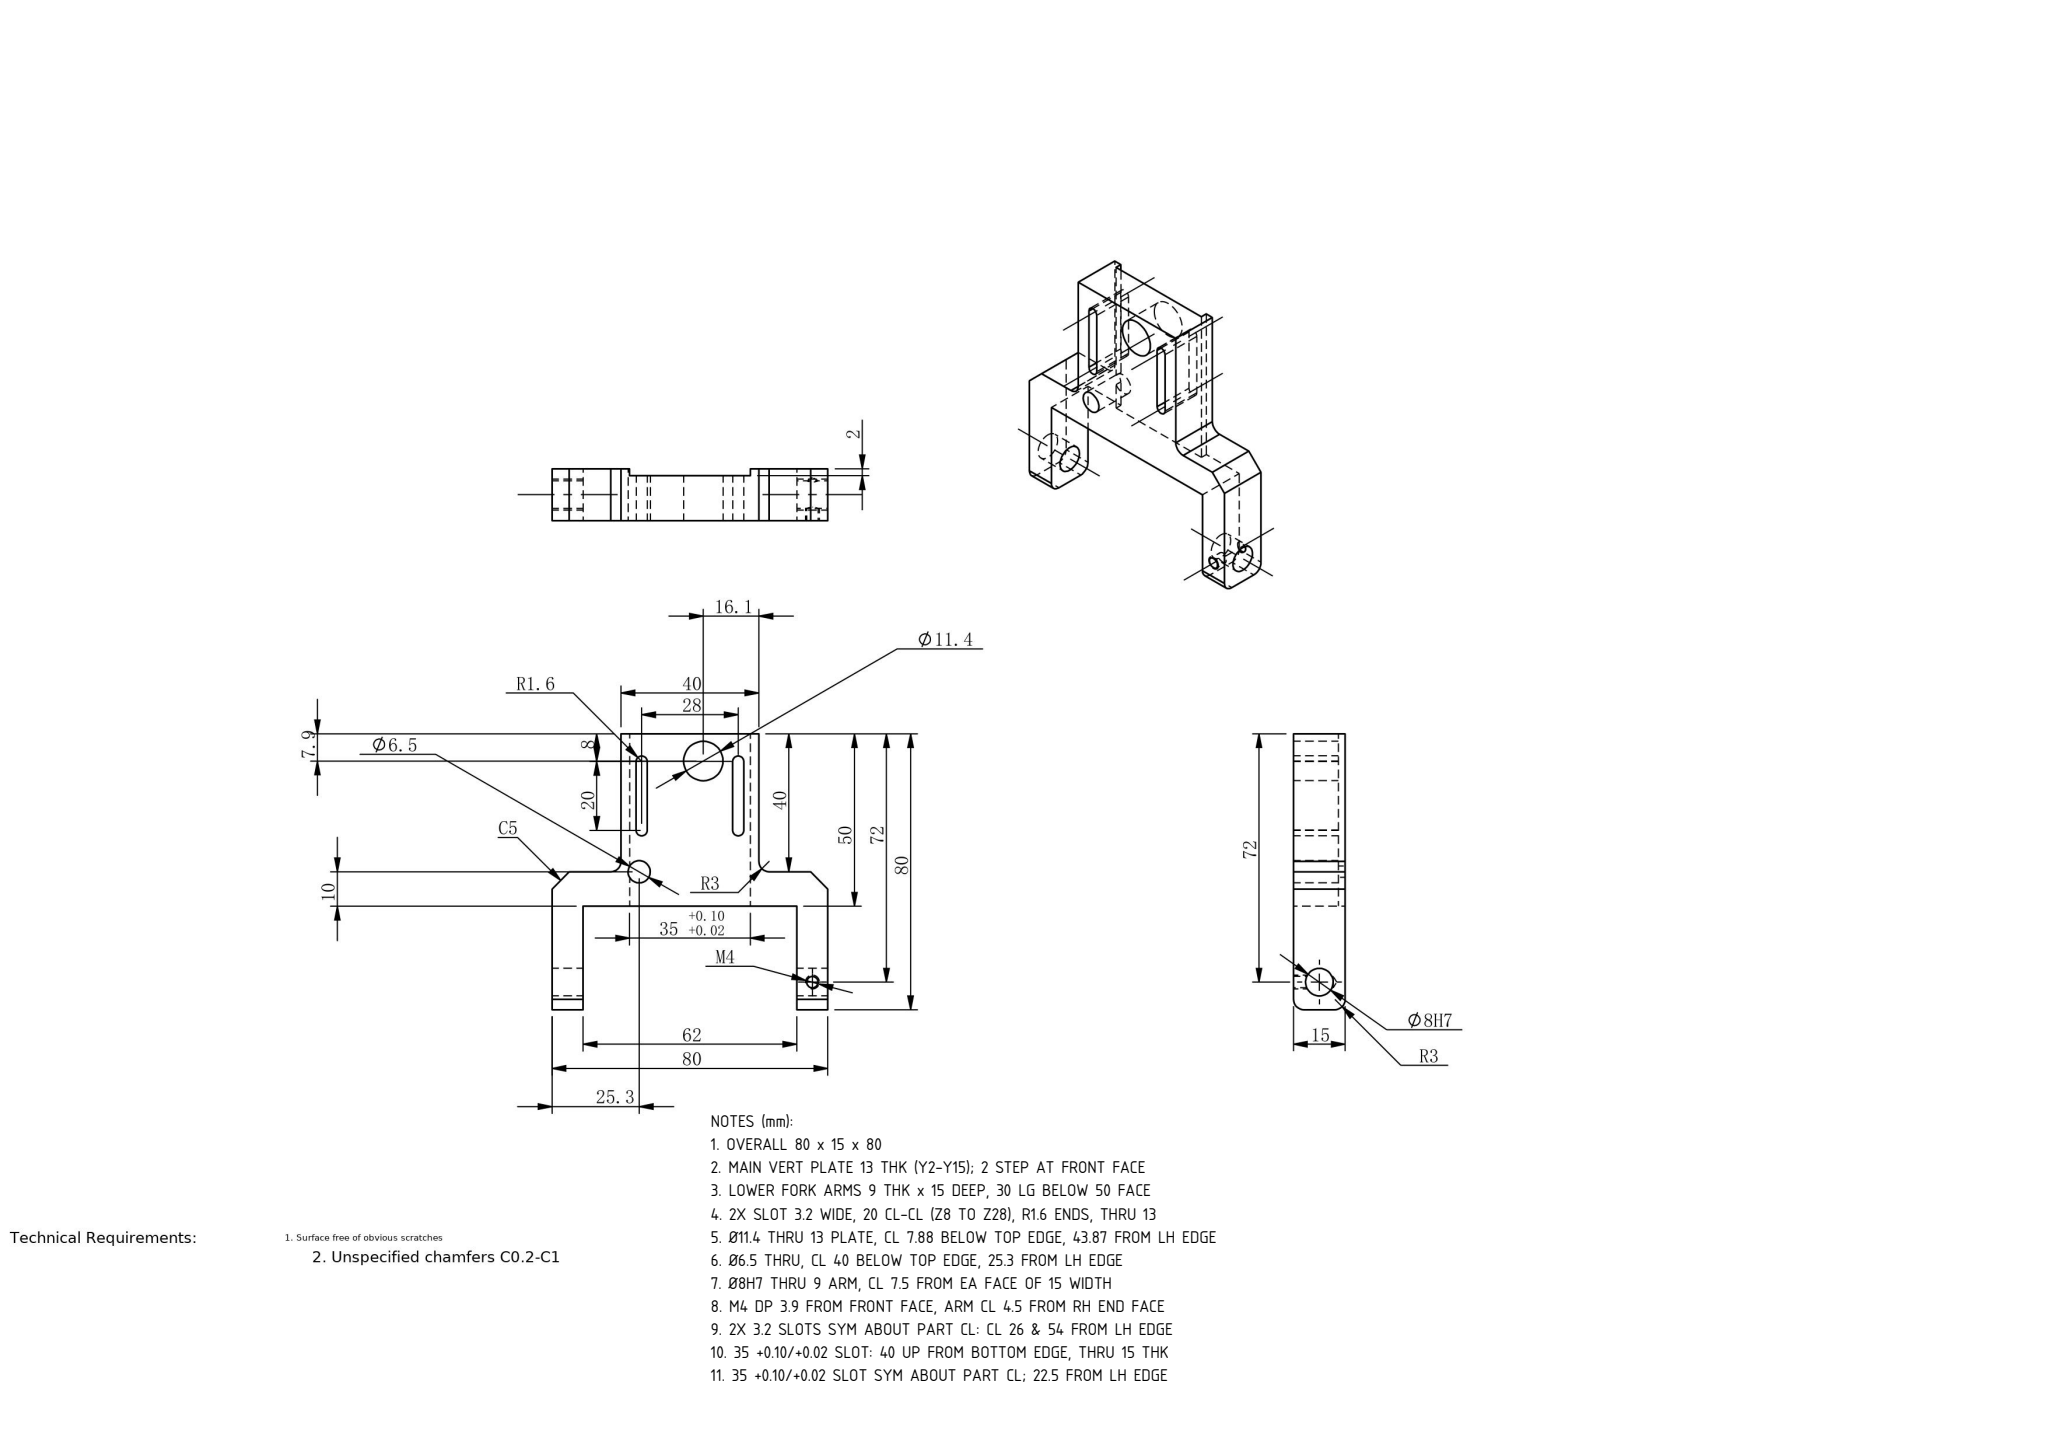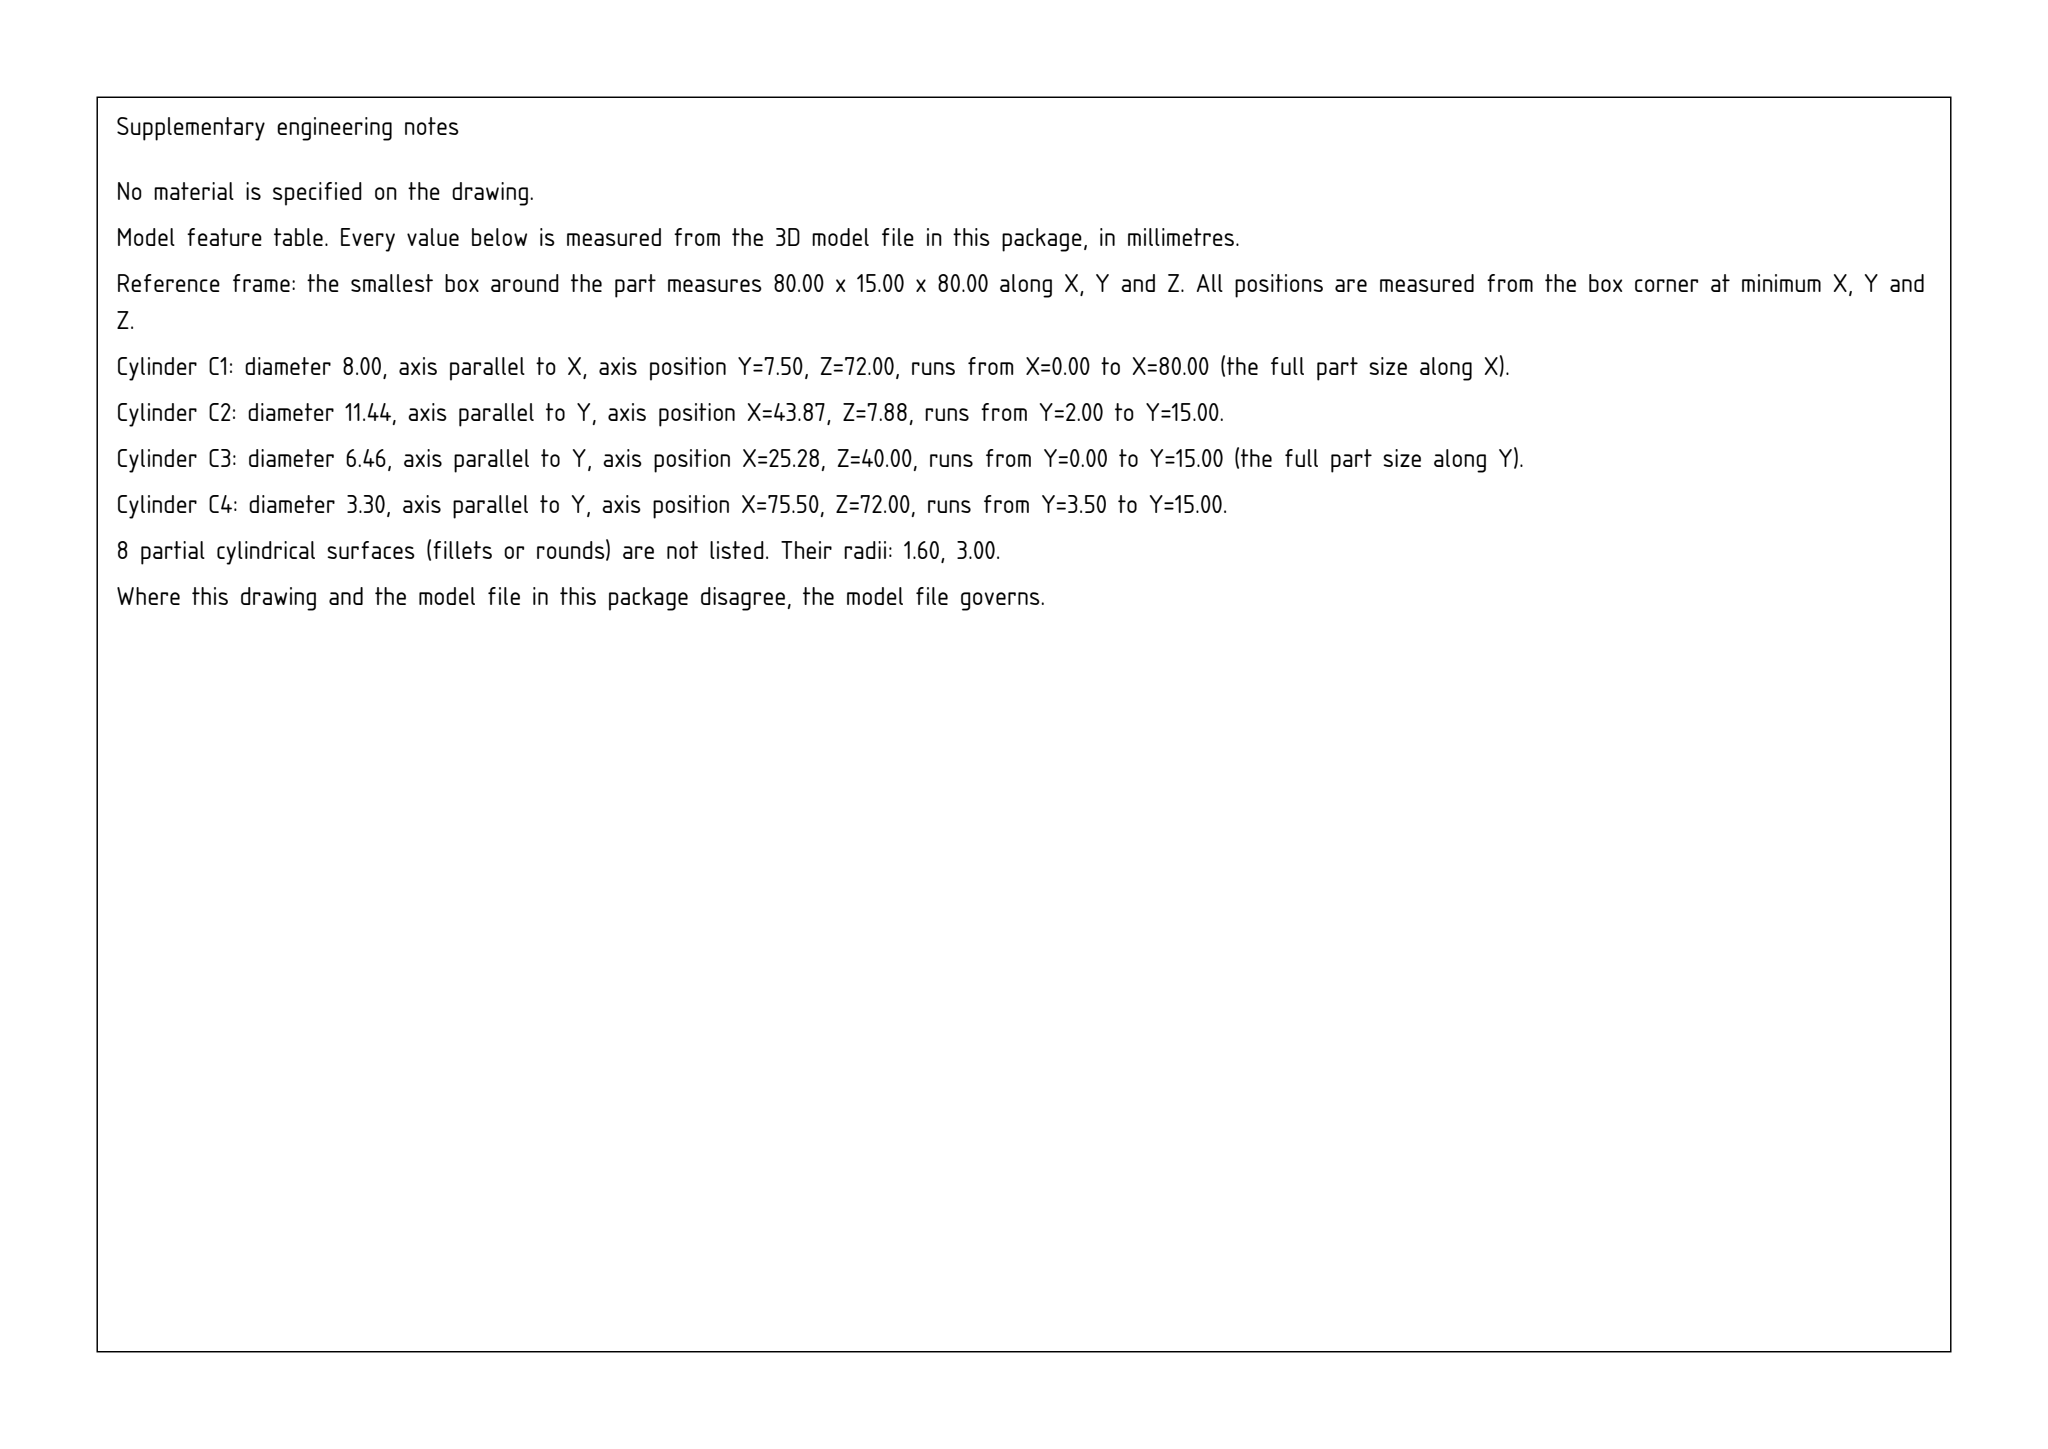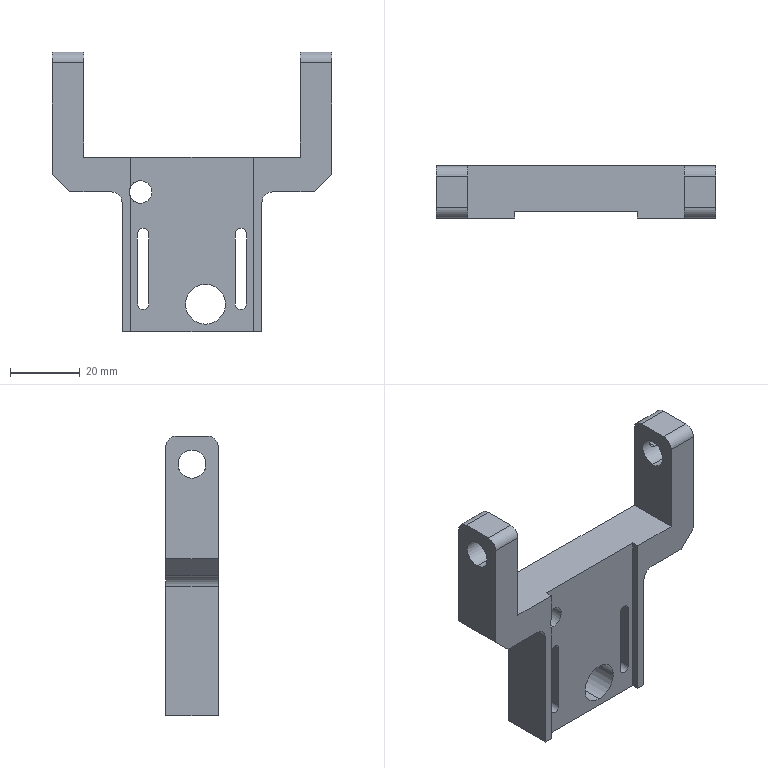Part | SolidWorks | mm | 1 solid | 52 faces | box 80 x 15 x 80 mm | volume 35640 mm3 | cylinder 25 | plane 25 | cone 2 | commonest cylinder face diameters 3.2 x6 6 x6 3.3 x5 8 x4 11.435 x2 6.45 x2
Drawing notes:
OVERALL 80 x 15 x 80 | from the solid: bbox_xyz 80,15,80
MAIN VERT PLATE 13 THK (Y2-Y15); 2 STEP AT FRONT FACE | from the solid: y-planes 0, 2, 15; plate holes 13 lg; bbox y=15
LOWER FORK ARMS 9 THK x 15 DEEP, 30 LG BELOW 50 FACE | from the solid: x-planes 0/9 and 71/80; z-planes 50 & 80; bbox y=15
2X SLOT 3.2 WIDE, 20 CL-CL (Z8 TO Z28), R1.6 ENDS, THRU 13 | from the solid: Ø3.2 axis y at x=26 & 54, z=8 & 28, len 13
Ø11.4 THRU 13 PLATE, CL 7.88 BELOW TOP EDGE, 43.87 FROM LH EDGE | from the solid: Ø11.435 axis y at [43.87, z=7.88], len 13
Ø6.5 THRU, CL 40 BELOW TOP EDGE, 25.3 FROM LH EDGE | from the solid: Ø6.45 axis y at x=25.28, z=40, len 13 & 15 = thru
Ø8H7 THRU 9 ARM, CL 7.5 FROM EA FACE OF 15 WIDTH | from the solid: Ø8 axis x at [y=7.5, z=72], len 9
M4 DP 3.9 FROM FRONT FACE, ARM CL 4.5 FROM RH END FACE | from the solid: Ø3.3 axis y at [75.5, z=72], len 3.86 + 118° tip; arm x71-80
2X 3.2 SLOTS SYM ABOUT PART CL: CL 26 & 54 FROM LH EDGE | from the solid: Ø3.2 y-axis cyls at x=26.0 and x=54.0 (bbox X=80, so sym about X=40); CL-CL 28
35 +0.10/+0.02 SLOT: 40 UP FROM BOTTOM EDGE, THRU 15 THK | from the solid: x-planes 22.5 & 57.5 (=35 wide), z-plane 40.0 slot top, y 0 to 15 full thk
35 +0.10/+0.02 SLOT SYM ABOUT PART CL; 22.5 FROM LH EDGE | from the solid: x-planes at 22.5 and 57.5 (2 faces) give 35 wide slot, centered on x=40 = half of 80 bbox width
build123d program:
from build123d import *

# Parameters (mm, degrees)
SKETCH1_W             = 80
SKETCH1_H             = 80
BOSS_EXTRUDE1_DEPTH   = 7.5
SKETCH2_W             = 62
SKETCH2_H             = 60
SKETCH2_W_2           = 20
SKETCH2_H_2           = 40
CUT_EXTRUDE1_DEPTH    = 59.523
FILLET1_R             = 3
FILLET2_R             = 3
CHAMFER1_SIZE         = 5
SKETCH3_W             = 35
SKETCH3_H             = 2
CUT_EXTRUDE2_DEPTH    = 90.757
CUT_EXTRUDE3_DEPTH    = 59.523
SKETCH5_R             = 4
CUT_EXTRUDE4_DEPTH    = 90.757
M4_TAPPED_HOLE1_D     = 3.3
M4_TAPPED_HOLE1_DEPTH = 11.5
M4_TAPPED_HOLE1_TIP   = 0.9914
SKETCH8_R             = 3.225
SKETCH8_R_2           = 5.717
CUT_EXTRUDE5_DEPTH    = 48


with BuildPart() as part:
    # Sketch1 → Boss-Extrude1 (new, symmetric)
    with BuildSketch(Plane(origin=(0, 0, 0), x_dir=(1, 0, 0), z_dir=(0, 1, 0))):
        Rectangle(SKETCH1_W, SKETCH1_H)
    extrude(amount=BOSS_EXTRUDE1_DEPTH, both=True)

    # Sketch2 → Cut-Extrude1 (cut, through all)
    with BuildSketch(Plane(origin=(0, 7.5, 0), x_dir=(1, 0, 0), z_dir=(0, 1, 0))):
        with Locations((0, -40)):
            Rectangle(SKETCH2_W, SKETCH2_H)
        with Locations((-30, 20)):
            Rectangle(SKETCH2_W_2, SKETCH2_H_2)
        with Locations((30, 20)):
            Rectangle(SKETCH2_W_2, SKETCH2_H_2)
    extrude(amount=-CUT_EXTRUDE1_DEPTH, mode=Mode.SUBTRACT)

    # Fillet1
    fillet1_edges = [part.edges().sort_by_distance(p)[0] for p in [
        (-35.5, 7.5, 40),
        (35.5, -7.5, 40),
        (35.5, 7.5, 40),
        (-35.5, -7.5, 40),
    ]]
    fillet(fillet1_edges, radius=FILLET1_R)

    # Fillet2
    fillet2_edges = [part.edges().sort_by_distance(p)[0] for p in [
        (-20, 0, 0),
        (20, 0, 0),
    ]]
    fillet(fillet2_edges, radius=FILLET2_R)

    # Chamfer1
    chamfer1_edges = [part.edges().sort_by_distance(p)[0] for p in [
        (-40, 0, 0),
        (40, 0, 0),
    ]]
    chamfer(chamfer1_edges, length=CHAMFER1_SIZE)

    # Sketch3 → Cut-Extrude2 (cut, through all)
    with BuildSketch(Plane(origin=(0, 0, -40), x_dir=(-1, 0, 0), z_dir=(0, 0, -1))):
        with Locations((0, -6.5)):
            Rectangle(SKETCH3_W, SKETCH3_H)
    extrude(amount=-CUT_EXTRUDE2_DEPTH, mode=Mode.SUBTRACT)

    # Sketch4 → Cut-Extrude3 (cut, through all)
    with BuildSketch(Plane(origin=(0, 7.5, 0), x_dir=(1, 0, 0), z_dir=(0, 1, 0))):
        with BuildLine():
            Line((15.6, 32), (15.6, 12))
            ThreePointArc((15.6, 12), (14, 10.4), (12.4, 12))
            Line((12.4, 12), (12.4, 32))
            ThreePointArc((12.4, 32), (14, 33.6), (15.6, 32))
        make_face()
        with BuildLine():
            Line((-12.4, 32), (-12.4, 12))
            ThreePointArc((-12.4, 12), (-14, 10.4), (-15.6, 12))
            Line((-15.6, 12), (-15.6, 32))
            ThreePointArc((-15.6, 32), (-14, 33.6), (-12.4, 32))
        make_face()
    extrude(amount=-CUT_EXTRUDE3_DEPTH, mode=Mode.SUBTRACT)

    # Sketch5 → Cut-Extrude4 (cut, through all)
    with BuildSketch(Plane(origin=(40, 0, 0), x_dir=(0, 0, -1), z_dir=(1, 0, 0))):
        with Locations((-32, 0)):
            Circle(SKETCH5_R)
    extrude(amount=-CUT_EXTRUDE4_DEPTH, mode=Mode.SUBTRACT)

    # M4 Tapped Hole1
    with Locations(Plane(origin=(0, 7.5, 0), x_dir=(-1, 0, 0), z_dir=(0, 1, 0))):
        with Locations((-35.5, 32)):
            Hole(M4_TAPPED_HOLE1_D / 2, depth=M4_TAPPED_HOLE1_DEPTH)
            with Locations((0, 0, -(M4_TAPPED_HOLE1_DEPTH + M4_TAPPED_HOLE1_TIP / 2))):  # 118° drill point
                Cone(0, M4_TAPPED_HOLE1_D / 2, M4_TAPPED_HOLE1_TIP, mode=Mode.SUBTRACT)

    # Sketch8 → Cut-Extrude5 (cut)
    with BuildSketch(Plane(origin=(0, 7.5, 0), x_dir=(1, 0, 0), z_dir=(0, 1, 0))):
        with Locations(Location((-14.723, 0, 0), (0, 0, 270))):
            Circle(SKETCH8_R)
        with Locations(Location((3.874, 32.119, 0), (0, 0, 270))):
            Circle(SKETCH8_R_2)
    extrude(amount=-CUT_EXTRUDE5_DEPTH, mode=Mode.SUBTRACT)


solid = part.part